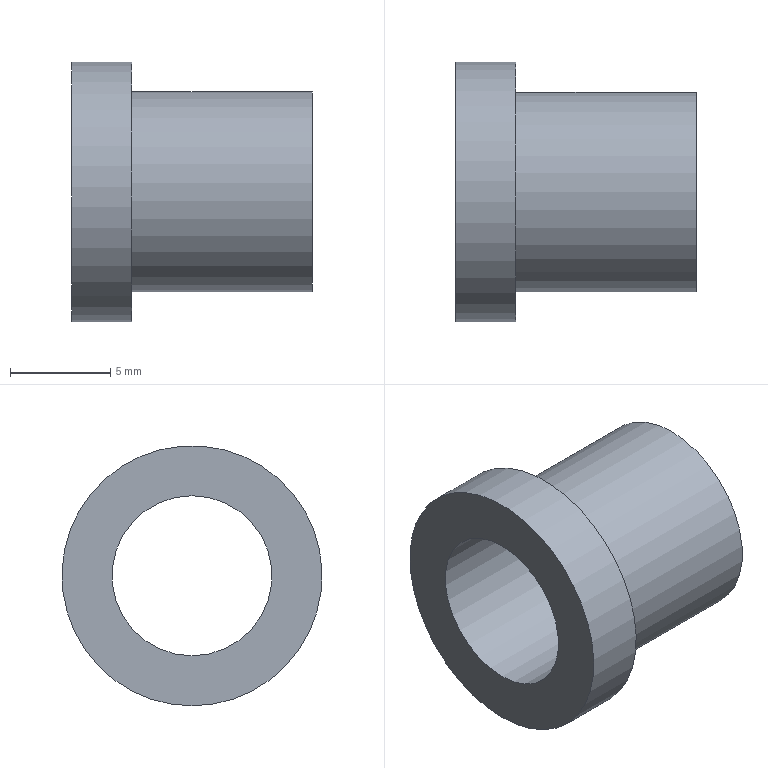Component | NX | ASSY_PRAC_PART_2 | 1 solid | 6 faces | box 12 x 13 x 13 mm | volume 502 mm3 | plane 3 | cylinder 3 | commonest cylinder face diameters 13 x1 10 x1 8 x1
STEP:
#1=CARTESIAN_POINT('',(0.,0.,0.));
#2=DIRECTION('',(0.,0.,1.));
#3=DIRECTION('',(1.,0.,0.));
#4=AXIS2_PLACEMENT_3D('',#1,#2,#3);
#5=CARTESIAN_POINT('',(-8.5,0.3851,16.561));
#6=VERTEX_POINT('',#5);
#7=CARTESIAN_POINT('',(-8.5,0.3851,20.561));
#8=DIRECTION('',(-1.,0.,0.));
#9=DIRECTION('',(0.,0.,-1.));
#10=AXIS2_PLACEMENT_3D('',#7,#8,#9);
#11=CIRCLE('',#10,4.);
#12=CARTESIAN_POINT('',(-8.5,-6.115,20.561));
#13=DIRECTION('',(1.,0.,0.));
#14=DIRECTION('',(0.,0.,1.));
#15=AXIS2_PLACEMENT_3D('',#12,#13,#14);
#16=PLANE('',#15);
#17=CARTESIAN_POINT('',(-4.,-6.5));
#18=CARTESIAN_POINT('',(-4.,0.4282));
#19=CARTESIAN_POINT('',(2.,-3.036));
#20=CARTESIAN_POINT('',(8.,-6.5));
#21=CARTESIAN_POINT('',(2.,-9.964));
#22=CARTESIAN_POINT('',(-4.,-13.428));
#23=CARTESIAN_POINT('',(-4.,-6.5));
#24=(BOUNDED_CURVE()B_SPLINE_CURVE(2,(#17,#18,#19,#20,#21,#22,#23),.UNSPECIFIED.,.T.,.F.)B_SPLINE_CURVE_WITH_KNOTS((1,2,2,2,2,1),(-2.094,0.,2.094,4.189,6.283,8.378),.UNSPECIFIED.)CURVE()GEOMETRIC_REPRESENTATION_ITEM()RATIONAL_B_SPLINE_CURVE((1.,0.5,1.,0.5,1.,0.5,1.))REPRESENTATION_ITEM(''));
#25=(GEOMETRIC_REPRESENTATION_CONTEXT(2)PARAMETRIC_REPRESENTATION_CONTEXT()REPRESENTATION_CONTEXT('',''));
#26=DEFINITIONAL_REPRESENTATION('',(#24),#25);
#27=PCURVE('',#16,#26);
#28=CARTESIAN_POINT('',(3.5,0.3851,20.561));
#29=DIRECTION('',(-1.,0.,0.));
#30=DIRECTION('',(0.,0.,-1.));
#31=AXIS2_PLACEMENT_3D('',#28,#29,#30);
#32=CYLINDRICAL_SURFACE('',#31,4.);
#33=CARTESIAN_POINT('',(0.,12.));
#34=DIRECTION('',(1.,0.));
#35=VECTOR('',#34,1.);
#36=LINE('',#33,#35);
#37=(GEOMETRIC_REPRESENTATION_CONTEXT(2)PARAMETRIC_REPRESENTATION_CONTEXT()REPRESENTATION_CONTEXT('',''));
#38=DEFINITIONAL_REPRESENTATION('',(#36),#37);
#39=PCURVE('',#32,#38);
#40=SURFACE_CURVE('',#11,(#27,#39),.PCURVE_S1.);
#41=EDGE_CURVE('',#6,#6,#40,.T.);
#42=ORIENTED_EDGE('',*,*,#41,.F.);
#43=EDGE_LOOP('',(#42));
#44=FACE_BOUND('',#43,.T.);
#45=CARTESIAN_POINT('',(-8.5,0.3851,14.061));
#46=VERTEX_POINT('',#45);
#47=CARTESIAN_POINT('',(-8.5,0.3851,20.561));
#48=DIRECTION('',(-1.,0.,0.));
#49=DIRECTION('',(0.,0.,-1.));
#50=AXIS2_PLACEMENT_3D('',#47,#48,#49);
#51=CIRCLE('',#50,6.5);
#52=CARTESIAN_POINT('',(-6.5,-6.5));
#53=CARTESIAN_POINT('',(-6.5,4.758));
#54=CARTESIAN_POINT('',(3.25,-0.8708));
#55=CARTESIAN_POINT('',(13.,-6.5));
#56=CARTESIAN_POINT('',(3.25,-12.129));
#57=CARTESIAN_POINT('',(-6.5,-17.758));
#58=CARTESIAN_POINT('',(-6.5,-6.5));
#59=(BOUNDED_CURVE()B_SPLINE_CURVE(2,(#52,#53,#54,#55,#56,#57,#58),.UNSPECIFIED.,.T.,.F.)B_SPLINE_CURVE_WITH_KNOTS((1,2,2,2,2,1),(-2.094,0.,2.094,4.189,6.283,8.378),.UNSPECIFIED.)CURVE()GEOMETRIC_REPRESENTATION_ITEM()RATIONAL_B_SPLINE_CURVE((1.,0.5,1.,0.5,1.,0.5,1.))REPRESENTATION_ITEM(''));
#60=(GEOMETRIC_REPRESENTATION_CONTEXT(2)PARAMETRIC_REPRESENTATION_CONTEXT()REPRESENTATION_CONTEXT('',''));
#61=DEFINITIONAL_REPRESENTATION('',(#59),#60);
#62=PCURVE('',#16,#61);
#63=CARTESIAN_POINT('',(3.5,0.3851,20.561));
#64=DIRECTION('',(-1.,0.,0.));
#65=DIRECTION('',(0.,0.,-1.));
#66=AXIS2_PLACEMENT_3D('',#63,#64,#65);
#67=CYLINDRICAL_SURFACE('',#66,6.5);
#68=CARTESIAN_POINT('',(0.,12.));
#69=DIRECTION('',(1.,0.));
#70=VECTOR('',#69,1.);
#71=LINE('',#68,#70);
#72=(GEOMETRIC_REPRESENTATION_CONTEXT(2)PARAMETRIC_REPRESENTATION_CONTEXT()REPRESENTATION_CONTEXT('',''));
#73=DEFINITIONAL_REPRESENTATION('',(#71),#72);
#74=PCURVE('',#67,#73);
#75=SURFACE_CURVE('',#51,(#62,#74),.PCURVE_S1.);
#76=EDGE_CURVE('',#46,#46,#75,.T.);
#77=ORIENTED_EDGE('',*,*,#76,.T.);
#78=EDGE_LOOP('',(#77));
#79=FACE_BOUND('',#78,.T.);
#80=ADVANCED_FACE('',(#44,#79),#16,.F.);
#81=ORIENTED_EDGE('',*,*,#76,.F.);
#82=CARTESIAN_POINT('',(-5.5,0.3851,14.061));
#83=VERTEX_POINT('',#82);
#84=CARTESIAN_POINT('',(-5.5,0.3851,14.061));
#85=CARTESIAN_POINT('',(-8.5,0.3851,14.061));
#86=B_SPLINE_CURVE_WITH_KNOTS('',1,(#84,#85),.UNSPECIFIED.,.F.,.F.,(2,2),(9.,12.),.PIECEWISE_BEZIER_KNOTS.);
#87=CARTESIAN_POINT('',(0.,0.));
#88=DIRECTION('',(0.,1.));
#89=VECTOR('',#88,1.);
#90=LINE('',#87,#89);
#91=(GEOMETRIC_REPRESENTATION_CONTEXT(2)PARAMETRIC_REPRESENTATION_CONTEXT()REPRESENTATION_CONTEXT('',''));
#92=DEFINITIONAL_REPRESENTATION('',(#90),#91);
#93=PCURVE('',#67,#92);
#94=CARTESIAN_POINT('',(6.283,0.));
#95=DIRECTION('',(0.,1.));
#96=VECTOR('',#95,1.);
#97=LINE('',#94,#96);
#98=(GEOMETRIC_REPRESENTATION_CONTEXT(2)PARAMETRIC_REPRESENTATION_CONTEXT()REPRESENTATION_CONTEXT('',''));
#99=DEFINITIONAL_REPRESENTATION('',(#97),#98);
#100=PCURVE('',#67,#99);
#101=SEAM_CURVE('',#86,(#93,#100),.PCURVE_S1.);
#102=EDGE_CURVE('',#83,#46,#101,.T.);
#103=ORIENTED_EDGE('',*,*,#102,.F.);
#104=CARTESIAN_POINT('',(-5.5,0.3851,20.561));
#105=DIRECTION('',(-1.,0.,0.));
#106=DIRECTION('',(0.,0.,-1.));
#107=AXIS2_PLACEMENT_3D('',#104,#105,#106);
#108=CIRCLE('',#107,6.5);
#109=CARTESIAN_POINT('',(0.,9.));
#110=DIRECTION('',(1.,0.));
#111=VECTOR('',#110,1.);
#112=LINE('',#109,#111);
#113=(GEOMETRIC_REPRESENTATION_CONTEXT(2)PARAMETRIC_REPRESENTATION_CONTEXT()REPRESENTATION_CONTEXT('',''));
#114=DEFINITIONAL_REPRESENTATION('',(#112),#113);
#115=PCURVE('',#67,#114);
#116=CARTESIAN_POINT('',(-5.5,-4.615,20.561));
#117=DIRECTION('',(-1.,0.,0.));
#118=DIRECTION('',(0.,0.,-1.));
#119=AXIS2_PLACEMENT_3D('',#116,#117,#118);
#120=PLANE('',#119);
#121=CARTESIAN_POINT('',(0.,-5.));
#122=DIRECTION('',(1.,0.));
#123=AXIS2_PLACEMENT_2D('',#121,#122);
#124=CIRCLE('',#123,6.5);
#125=(GEOMETRIC_REPRESENTATION_CONTEXT(2)PARAMETRIC_REPRESENTATION_CONTEXT()REPRESENTATION_CONTEXT('',''));
#126=DEFINITIONAL_REPRESENTATION('',(#124),#125);
#127=PCURVE('',#120,#126);
#128=SURFACE_CURVE('',#108,(#115,#127),.PCURVE_S1.);
#129=EDGE_CURVE('',#83,#83,#128,.T.);
#130=ORIENTED_EDGE('',*,*,#129,.T.);
#131=ORIENTED_EDGE('',*,*,#102,.T.);
#132=EDGE_LOOP('',(#81,#103,#130,#131));
#133=FACE_BOUND('',#132,.T.);
#134=ADVANCED_FACE('',(#133),#67,.T.);
#135=ORIENTED_EDGE('',*,*,#129,.F.);
#136=EDGE_LOOP('',(#135));
#137=FACE_BOUND('',#136,.T.);
#138=CARTESIAN_POINT('',(-5.5,0.3851,15.561));
#139=VERTEX_POINT('',#138);
#140=CARTESIAN_POINT('',(-5.5,0.3851,20.561));
#141=DIRECTION('',(-1.,0.,0.));
#142=DIRECTION('',(0.,0.,-1.));
#143=AXIS2_PLACEMENT_3D('',#140,#141,#142);
#144=CIRCLE('',#143,5.);
#145=CARTESIAN_POINT('',(0.,-5.));
#146=DIRECTION('',(1.,0.));
#147=AXIS2_PLACEMENT_2D('',#145,#146);
#148=CIRCLE('',#147,5.);
#149=(GEOMETRIC_REPRESENTATION_CONTEXT(2)PARAMETRIC_REPRESENTATION_CONTEXT()REPRESENTATION_CONTEXT('',''));
#150=DEFINITIONAL_REPRESENTATION('',(#148),#149);
#151=PCURVE('',#120,#150);
#152=CARTESIAN_POINT('',(3.5,0.3851,20.561));
#153=DIRECTION('',(-1.,0.,0.));
#154=DIRECTION('',(0.,0.,-1.));
#155=AXIS2_PLACEMENT_3D('',#152,#153,#154);
#156=CYLINDRICAL_SURFACE('',#155,5.);
#157=CARTESIAN_POINT('',(0.,9.));
#158=DIRECTION('',(1.,0.));
#159=VECTOR('',#158,1.);
#160=LINE('',#157,#159);
#161=(GEOMETRIC_REPRESENTATION_CONTEXT(2)PARAMETRIC_REPRESENTATION_CONTEXT()REPRESENTATION_CONTEXT('',''));
#162=DEFINITIONAL_REPRESENTATION('',(#160),#161);
#163=PCURVE('',#156,#162);
#164=SURFACE_CURVE('',#144,(#151,#163),.PCURVE_S1.);
#165=EDGE_CURVE('',#139,#139,#164,.T.);
#166=ORIENTED_EDGE('',*,*,#165,.T.);
#167=EDGE_LOOP('',(#166));
#168=FACE_BOUND('',#167,.T.);
#169=ADVANCED_FACE('',(#137,#168),#120,.F.);
#170=ORIENTED_EDGE('',*,*,#165,.F.);
#171=CARTESIAN_POINT('',(3.5,0.3851,15.561));
#172=VERTEX_POINT('',#171);
#173=CARTESIAN_POINT('',(3.5,0.3851,15.561));
#174=CARTESIAN_POINT('',(-5.5,0.3851,15.561));
#175=B_SPLINE_CURVE_WITH_KNOTS('',1,(#173,#174),.UNSPECIFIED.,.F.,.F.,(2,2),(0.,9.),.PIECEWISE_BEZIER_KNOTS.);
#176=CARTESIAN_POINT('',(0.,0.));
#177=DIRECTION('',(0.,1.));
#178=VECTOR('',#177,1.);
#179=LINE('',#176,#178);
#180=(GEOMETRIC_REPRESENTATION_CONTEXT(2)PARAMETRIC_REPRESENTATION_CONTEXT()REPRESENTATION_CONTEXT('',''));
#181=DEFINITIONAL_REPRESENTATION('',(#179),#180);
#182=PCURVE('',#156,#181);
#183=CARTESIAN_POINT('',(6.283,0.));
#184=DIRECTION('',(0.,1.));
#185=VECTOR('',#184,1.);
#186=LINE('',#183,#185);
#187=(GEOMETRIC_REPRESENTATION_CONTEXT(2)PARAMETRIC_REPRESENTATION_CONTEXT()REPRESENTATION_CONTEXT('',''));
#188=DEFINITIONAL_REPRESENTATION('',(#186),#187);
#189=PCURVE('',#156,#188);
#190=SEAM_CURVE('',#175,(#182,#189),.PCURVE_S1.);
#191=EDGE_CURVE('',#172,#139,#190,.T.);
#192=ORIENTED_EDGE('',*,*,#191,.F.);
#193=CARTESIAN_POINT('',(3.5,0.3851,20.561));
#194=DIRECTION('',(-1.,0.,0.));
#195=DIRECTION('',(0.,0.,-1.));
#196=AXIS2_PLACEMENT_3D('',#193,#194,#195);
#197=CIRCLE('',#196,5.);
#198=CARTESIAN_POINT('',(0.,0.));
#199=DIRECTION('',(1.,0.));
#200=VECTOR('',#199,1.);
#201=LINE('',#198,#200);
#202=(GEOMETRIC_REPRESENTATION_CONTEXT(2)PARAMETRIC_REPRESENTATION_CONTEXT()REPRESENTATION_CONTEXT('',''));
#203=DEFINITIONAL_REPRESENTATION('',(#201),#202);
#204=PCURVE('',#156,#203);
#205=CARTESIAN_POINT('',(3.5,0.3851,20.561));
#206=DIRECTION('',(-1.,0.,0.));
#207=DIRECTION('',(0.,0.,-1.));
#208=AXIS2_PLACEMENT_3D('',#205,#206,#207);
#209=PLANE('',#208);
#210=CARTESIAN_POINT('',(0.,0.));
#211=DIRECTION('',(1.,0.));
#212=AXIS2_PLACEMENT_2D('',#210,#211);
#213=CIRCLE('',#212,5.);
#214=(GEOMETRIC_REPRESENTATION_CONTEXT(2)PARAMETRIC_REPRESENTATION_CONTEXT()REPRESENTATION_CONTEXT('',''));
#215=DEFINITIONAL_REPRESENTATION('',(#213),#214);
#216=PCURVE('',#209,#215);
#217=SURFACE_CURVE('',#197,(#204,#216),.PCURVE_S1.);
#218=EDGE_CURVE('',#172,#172,#217,.T.);
#219=ORIENTED_EDGE('',*,*,#218,.T.);
#220=ORIENTED_EDGE('',*,*,#191,.T.);
#221=EDGE_LOOP('',(#170,#192,#219,#220));
#222=FACE_BOUND('',#221,.T.);
#223=ADVANCED_FACE('',(#222),#156,.T.);
#224=CARTESIAN_POINT('',(3.5,0.3851,16.561));
#225=VERTEX_POINT('',#224);
#226=CARTESIAN_POINT('',(3.5,0.3851,20.561));
#227=DIRECTION('',(-1.,0.,0.));
#228=DIRECTION('',(0.,0.,-1.));
#229=AXIS2_PLACEMENT_3D('',#226,#227,#228);
#230=CIRCLE('',#229,4.);
#231=CARTESIAN_POINT('',(0.,0.));
#232=DIRECTION('',(1.,0.));
#233=AXIS2_PLACEMENT_2D('',#231,#232);
#234=CIRCLE('',#233,4.);
#235=(GEOMETRIC_REPRESENTATION_CONTEXT(2)PARAMETRIC_REPRESENTATION_CONTEXT()REPRESENTATION_CONTEXT('',''));
#236=DEFINITIONAL_REPRESENTATION('',(#234),#235);
#237=PCURVE('',#209,#236);
#238=CARTESIAN_POINT('',(0.,0.));
#239=DIRECTION('',(1.,0.));
#240=VECTOR('',#239,1.);
#241=LINE('',#238,#240);
#242=(GEOMETRIC_REPRESENTATION_CONTEXT(2)PARAMETRIC_REPRESENTATION_CONTEXT()REPRESENTATION_CONTEXT('',''));
#243=DEFINITIONAL_REPRESENTATION('',(#241),#242);
#244=PCURVE('',#32,#243);
#245=SURFACE_CURVE('',#230,(#237,#244),.PCURVE_S1.);
#246=EDGE_CURVE('',#225,#225,#245,.T.);
#247=ORIENTED_EDGE('',*,*,#246,.T.);
#248=EDGE_LOOP('',(#247));
#249=FACE_BOUND('',#248,.T.);
#250=ORIENTED_EDGE('',*,*,#218,.F.);
#251=EDGE_LOOP('',(#250));
#252=FACE_BOUND('',#251,.T.);
#253=ADVANCED_FACE('',(#249,#252),#209,.F.);
#254=ORIENTED_EDGE('',*,*,#41,.F.);
#255=CARTESIAN_POINT('',(3.5,0.3851,16.561));
#256=CARTESIAN_POINT('',(-8.5,0.3851,16.561));
#257=B_SPLINE_CURVE_WITH_KNOTS('',1,(#255,#256),.UNSPECIFIED.,.F.,.F.,(2,2),(0.,12.),.PIECEWISE_BEZIER_KNOTS.);
#258=CARTESIAN_POINT('',(0.,0.));
#259=DIRECTION('',(0.,1.));
#260=VECTOR('',#259,1.);
#261=LINE('',#258,#260);
#262=(GEOMETRIC_REPRESENTATION_CONTEXT(2)PARAMETRIC_REPRESENTATION_CONTEXT()REPRESENTATION_CONTEXT('',''));
#263=DEFINITIONAL_REPRESENTATION('',(#261),#262);
#264=PCURVE('',#32,#263);
#265=CARTESIAN_POINT('',(6.283,0.));
#266=DIRECTION('',(0.,1.));
#267=VECTOR('',#266,1.);
#268=LINE('',#265,#267);
#269=(GEOMETRIC_REPRESENTATION_CONTEXT(2)PARAMETRIC_REPRESENTATION_CONTEXT()REPRESENTATION_CONTEXT('',''));
#270=DEFINITIONAL_REPRESENTATION('',(#268),#269);
#271=PCURVE('',#32,#270);
#272=SEAM_CURVE('',#257,(#264,#271),.PCURVE_S1.);
#273=EDGE_CURVE('',#225,#6,#272,.T.);
#274=ORIENTED_EDGE('',*,*,#273,.F.);
#275=ORIENTED_EDGE('',*,*,#246,.T.);
#276=ORIENTED_EDGE('',*,*,#273,.T.);
#277=EDGE_LOOP('',(#254,#274,#275,#276));
#278=FACE_BOUND('',#277,.F.);
#279=ADVANCED_FACE('',(#278),#32,.F.);
#280=CLOSED_SHELL('',(#80,#134,#169,#223,#253,#279));
#281=MANIFOLD_SOLID_BREP('',#280);
#282=(LENGTH_UNIT()NAMED_UNIT(*)SI_UNIT(.MILLI.,.METRE.));
#283=UNCERTAINTY_MEASURE_WITH_UNIT(LENGTH_MEASURE(0.00001),#282,'','');
#284=(NAMED_UNIT(*)PLANE_ANGLE_UNIT()SI_UNIT($,.RADIAN.));
#285=(NAMED_UNIT(*)SI_UNIT($,.STERADIAN.)SOLID_ANGLE_UNIT());
#286=(GEOMETRIC_REPRESENTATION_CONTEXT(3)GLOBAL_UNCERTAINTY_ASSIGNED_CONTEXT((#283))GLOBAL_UNIT_ASSIGNED_CONTEXT((#282,#284,#285))REPRESENTATION_CONTEXT('',''));
#287=ADVANCED_BREP_SHAPE_REPRESENTATION('',(#4,#281),#286);